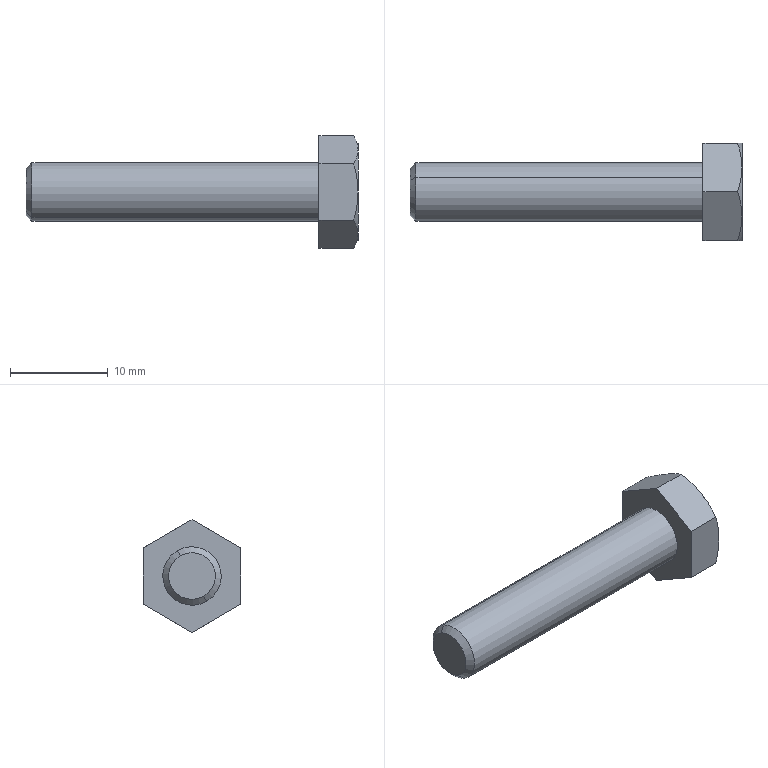Component | SolidWorks | Q1-A12-S21-Q1D.SLDASQ-1_Q1-RCB6-30-1 | 1 solid | 19 faces | box 34 x 10 x 11.55 mm | volume 1190 mm3 | plane 9 | cone 8 | cylinder 2 | commonest cylinder face diameters 6 x2
build123d program:
from build123d import *

# Parameters (mm, degrees)
SKETCH2_W          = 20
SKETCH2_H          = 20
CUT_EXTRUDE1_DEPTH = 4


with BuildPart() as part:
    # Sketch1 → Revolve1 (revolve)
    with BuildSketch(Plane.XY, mode=Mode.PRIVATE) as revolve1_sk:
        Polygon((-4, 0), (-4, 5), (-3.423, 6), (0, 6), (0, 3), (29.387, 3), (30, 2.386), (30, 0), align=None)
    revolve(revolve1_sk.sketch.rotate(Axis((30, 0, 0), (-1, 0, 0)), 270), axis=Axis((30, 0, 0), (-1, 0, 0)))

    # Sketch2 → Cut-Extrude1 (cut)
    with BuildSketch(Plane(origin=(-4, 0, 0), x_dir=(0, 0, -1), z_dir=(1, 0, 0))):
        Rectangle(SKETCH2_W, SKETCH2_H)
        Polygon((-5, -2.887), (0, -5.774), (5, -2.887), (5, 2.887), (0, 5.774), (-5, 2.887), align=None, mode=Mode.SUBTRACT)
    extrude(amount=CUT_EXTRUDE1_DEPTH, mode=Mode.SUBTRACT)


solid = part.part

# Placed as in the assembly
solid = solid.moved(Location((1985.5, 0, 156.25), (-90, 0, 180)))
STEP:
#1=COLOUR_RGB('',0.7922,0.8196,0.9333);
#2=FILL_AREA_STYLE_COLOUR('',#1);
#3=FILL_AREA_STYLE('',(#2));
#4=SURFACE_STYLE_FILL_AREA(#3);
#5=SURFACE_SIDE_STYLE('',(#4));
#6=SURFACE_STYLE_USAGE(.BOTH.,#5);
#7=PRESENTATION_STYLE_ASSIGNMENT((#6));
#8=CARTESIAN_POINT('',(76.988,-0.04698,6.07));
#9=VERTEX_POINT('',#8);
#10=CARTESIAN_POINT('',(76.988,0.04698,6.233));
#11=VERTEX_POINT('',#10);
#12=CARTESIAN_POINT('',(76.988,0.,6.152));
#13=DIRECTION('',(1.,-0.,-0.));
#14=DIRECTION('',(0.,-0.5,-0.866));
#15=AXIS2_PLACEMENT_3D('',#12,#13,#14);
#16=CIRCLE('',#15,0.09396);
#17=EDGE_CURVE('',#9,#11,#16,.T.);
#18=ORIENTED_EDGE('',*,*,#17,.T.);
#19=CARTESIAN_POINT('',(77.012,0.05906,6.254));
#20=VERTEX_POINT('',#19);
#21=CARTESIAN_POINT('',(76.988,0.04698,6.233));
#22=DIRECTION('',(0.7071,0.3536,0.6124));
#23=VECTOR('',#22,39.37);
#24=LINE('',#21,#23);
#25=EDGE_CURVE('',#11,#20,#24,.T.);
#26=ORIENTED_EDGE('',*,*,#25,.T.);
#27=CARTESIAN_POINT('',(77.012,-0.05906,6.049));
#28=VERTEX_POINT('',#27);
#29=CARTESIAN_POINT('',(77.012,0.,6.152));
#30=DIRECTION('',(1.,-0.,-0.));
#31=DIRECTION('',(0.,-0.5,-0.866));
#32=AXIS2_PLACEMENT_3D('',#29,#30,#31);
#33=CIRCLE('',#32,0.1181);
#34=EDGE_CURVE('',#28,#20,#33,.T.);
#35=ORIENTED_EDGE('',*,*,#34,.F.);
#36=CARTESIAN_POINT('',(76.988,-0.04698,6.07));
#37=DIRECTION('',(0.7071,-0.3536,-0.6124));
#38=VECTOR('',#37,39.37);
#39=LINE('',#36,#38);
#40=EDGE_CURVE('',#9,#28,#39,.T.);
#41=ORIENTED_EDGE('',*,*,#40,.F.);
#42=EDGE_LOOP('',(#18,#26,#35,#41));
#43=FACE_OUTER_BOUND('',#42,.T.);
#44=CARTESIAN_POINT('',(76.988,0.,6.152));
#45=DIRECTION('',(1.,-0.,-0.));
#46=DIRECTION('',(0.,-0.5,-0.866));
#47=AXIS2_PLACEMENT_3D('',#44,#45,#46);
#48=CONICAL_SURFACE('',#47,0.09396,0.7854);
#49=ADVANCED_FACE('',(#43),#48,.T.);
#50=ORIENTED_EDGE('',*,*,#34,.T.);
#51=CARTESIAN_POINT('',(78.169,0.05906,6.254));
#52=VERTEX_POINT('',#51);
#53=CARTESIAN_POINT('',(76.988,0.05906,6.254));
#54=DIRECTION('',(1.,-0.,-0.));
#55=VECTOR('',#54,39.37);
#56=LINE('',#53,#55);
#57=EDGE_CURVE('',#20,#52,#56,.T.);
#58=ORIENTED_EDGE('',*,*,#57,.T.);
#59=CARTESIAN_POINT('',(78.169,-0.05906,6.049));
#60=VERTEX_POINT('',#59);
#61=CARTESIAN_POINT('',(78.169,0.,6.152));
#62=DIRECTION('',(1.,-0.,-0.));
#63=DIRECTION('',(0.,-0.5,-0.866));
#64=AXIS2_PLACEMENT_3D('',#61,#62,#63);
#65=CIRCLE('',#64,0.1181);
#66=EDGE_CURVE('',#60,#52,#65,.T.);
#67=ORIENTED_EDGE('',*,*,#66,.F.);
#68=CARTESIAN_POINT('',(76.988,-0.05906,6.049));
#69=DIRECTION('',(1.,-0.,-0.));
#70=VECTOR('',#69,39.37);
#71=LINE('',#68,#70);
#72=EDGE_CURVE('',#28,#60,#71,.T.);
#73=ORIENTED_EDGE('',*,*,#72,.F.);
#74=EDGE_LOOP('',(#50,#58,#67,#73));
#75=FACE_OUTER_BOUND('',#74,.T.);
#76=CARTESIAN_POINT('',(76.988,0.,6.152));
#77=DIRECTION('',(1.,-0.,-0.));
#78=DIRECTION('',(0.,-0.5,-0.866));
#79=AXIS2_PLACEMENT_3D('',#76,#77,#78);
#80=CYLINDRICAL_SURFACE('',#79,0.1181);
#81=ADVANCED_FACE('',(#75),#80,.T.);
#82=CARTESIAN_POINT('',(78.169,0.1969,6.038));
#83=VERTEX_POINT('',#82);
#84=CARTESIAN_POINT('',(78.169,0.,5.924));
#85=VERTEX_POINT('',#84);
#86=CARTESIAN_POINT('',(78.169,0.1969,6.038));
#87=DIRECTION('',(-0.,-0.866,-0.5));
#88=VECTOR('',#87,39.37);
#89=LINE('',#86,#88);
#90=EDGE_CURVE('',#83,#85,#89,.T.);
#91=ORIENTED_EDGE('',*,*,#90,.T.);
#92=CARTESIAN_POINT('',(78.169,-0.1969,6.038));
#93=VERTEX_POINT('',#92);
#94=CARTESIAN_POINT('',(78.169,0.,5.924));
#95=DIRECTION('',(-0.,-0.866,0.5));
#96=VECTOR('',#95,39.37);
#97=LINE('',#94,#96);
#98=EDGE_CURVE('',#85,#93,#97,.T.);
#99=ORIENTED_EDGE('',*,*,#98,.T.);
#100=CARTESIAN_POINT('',(78.169,-0.1969,6.265));
#101=VERTEX_POINT('',#100);
#102=CARTESIAN_POINT('',(78.169,-0.1969,6.038));
#103=DIRECTION('',(-0.,-0.,1.));
#104=VECTOR('',#103,39.37);
#105=LINE('',#102,#104);
#106=EDGE_CURVE('',#93,#101,#105,.T.);
#107=ORIENTED_EDGE('',*,*,#106,.T.);
#108=CARTESIAN_POINT('',(78.169,0.,6.379));
#109=VERTEX_POINT('',#108);
#110=CARTESIAN_POINT('',(78.169,-0.1969,6.265));
#111=DIRECTION('',(0.,0.866,0.5));
#112=VECTOR('',#111,39.37);
#113=LINE('',#110,#112);
#114=EDGE_CURVE('',#101,#109,#113,.T.);
#115=ORIENTED_EDGE('',*,*,#114,.T.);
#116=CARTESIAN_POINT('',(78.169,0.1969,6.265));
#117=VERTEX_POINT('',#116);
#118=CARTESIAN_POINT('',(78.169,0.,6.379));
#119=DIRECTION('',(0.,0.866,-0.5));
#120=VECTOR('',#119,39.37);
#121=LINE('',#118,#120);
#122=EDGE_CURVE('',#109,#117,#121,.T.);
#123=ORIENTED_EDGE('',*,*,#122,.T.);
#124=CARTESIAN_POINT('',(78.169,0.1969,6.265));
#125=DIRECTION('',(0.,0.,-1.));
#126=VECTOR('',#125,39.37);
#127=LINE('',#124,#126);
#128=EDGE_CURVE('',#117,#83,#127,.T.);
#129=ORIENTED_EDGE('',*,*,#128,.T.);
#130=EDGE_LOOP('',(#91,#99,#107,#115,#123,#129));
#131=FACE_OUTER_BOUND('',#130,.T.);
#132=ORIENTED_EDGE('',*,*,#66,.T.);
#133=CARTESIAN_POINT('',(78.169,0.,6.152));
#134=DIRECTION('',(1.,-0.,-0.));
#135=DIRECTION('',(0.,-0.5,-0.866));
#136=AXIS2_PLACEMENT_3D('',#133,#134,#135);
#137=CIRCLE('',#136,0.1181);
#138=EDGE_CURVE('',#52,#60,#137,.T.);
#139=ORIENTED_EDGE('',*,*,#138,.T.);
#140=EDGE_LOOP('',(#132,#139));
#141=FACE_BOUND('',#140,.T.);
#142=CARTESIAN_POINT('',(78.169,0.2046,6.033));
#143=DIRECTION('',(1.,-0.,0.));
#144=DIRECTION('',(-0.,-0.5,-0.866));
#145=AXIS2_PLACEMENT_3D('',#142,#143,#144);
#146=PLANE('',#145);
#147=ADVANCED_FACE('',(#131,#141),#146,.F.);
#148=ORIENTED_EDGE('',*,*,#57,.F.);
#149=CARTESIAN_POINT('',(77.012,0.,6.152));
#150=DIRECTION('',(1.,-0.,-0.));
#151=DIRECTION('',(0.,-0.5,-0.866));
#152=AXIS2_PLACEMENT_3D('',#149,#150,#151);
#153=CIRCLE('',#152,0.1181);
#154=EDGE_CURVE('',#20,#28,#153,.T.);
#155=ORIENTED_EDGE('',*,*,#154,.T.);
#156=ORIENTED_EDGE('',*,*,#72,.T.);
#157=ORIENTED_EDGE('',*,*,#138,.F.);
#158=EDGE_LOOP('',(#148,#155,#156,#157));
#159=FACE_OUTER_BOUND('',#158,.T.);
#160=CARTESIAN_POINT('',(76.988,0.,6.152));
#161=DIRECTION('',(1.,-0.,-0.));
#162=DIRECTION('',(0.,-0.5,-0.866));
#163=AXIS2_PLACEMENT_3D('',#160,#161,#162);
#164=CYLINDRICAL_SURFACE('',#163,0.1181);
#165=ADVANCED_FACE('',(#159),#164,.T.);
#166=ORIENTED_EDGE('',*,*,#25,.F.);
#167=CARTESIAN_POINT('',(76.988,0.,6.152));
#168=DIRECTION('',(1.,-0.,-0.));
#169=DIRECTION('',(0.,-0.5,-0.866));
#170=AXIS2_PLACEMENT_3D('',#167,#168,#169);
#171=CIRCLE('',#170,0.09396);
#172=EDGE_CURVE('',#11,#9,#171,.T.);
#173=ORIENTED_EDGE('',*,*,#172,.T.);
#174=ORIENTED_EDGE('',*,*,#40,.T.);
#175=ORIENTED_EDGE('',*,*,#154,.F.);
#176=EDGE_LOOP('',(#166,#173,#174,#175));
#177=FACE_OUTER_BOUND('',#176,.T.);
#178=CARTESIAN_POINT('',(76.988,0.,6.152));
#179=DIRECTION('',(1.,-0.,-0.));
#180=DIRECTION('',(0.,-0.5,-0.866));
#181=AXIS2_PLACEMENT_3D('',#178,#179,#180);
#182=CONICAL_SURFACE('',#181,0.09396,0.7854);
#183=ADVANCED_FACE('',(#177),#182,.T.);
#184=ORIENTED_EDGE('',*,*,#17,.F.);
#185=ORIENTED_EDGE('',*,*,#172,.F.);
#186=EDGE_LOOP('',(#184,#185));
#187=FACE_OUTER_BOUND('',#186,.T.);
#188=CARTESIAN_POINT('',(76.988,0.08137,6.105));
#189=DIRECTION('',(1.,-0.,0.));
#190=DIRECTION('',(-0.,-0.5,-0.866));
#191=AXIS2_PLACEMENT_3D('',#188,#189,#190);
#192=PLANE('',#191);
#193=ADVANCED_FACE('',(#187),#192,.F.);
#194=CARTESIAN_POINT('',(78.309,-0.1969,6.038));
#195=VERTEX_POINT('',#194);
#196=CARTESIAN_POINT('',(78.169,-0.1969,6.038));
#197=DIRECTION('',(1.,-0.,-0.));
#198=VECTOR('',#197,39.37);
#199=LINE('',#196,#198);
#200=EDGE_CURVE('',#93,#195,#199,.T.);
#201=ORIENTED_EDGE('',*,*,#200,.F.);
#202=ORIENTED_EDGE('',*,*,#98,.F.);
#203=CARTESIAN_POINT('',(78.309,0.,5.924));
#204=VERTEX_POINT('',#203);
#205=CARTESIAN_POINT('',(78.169,0.,5.924));
#206=DIRECTION('',(1.,-0.,-0.));
#207=VECTOR('',#206,39.37);
#208=LINE('',#205,#207);
#209=EDGE_CURVE('',#85,#204,#208,.T.);
#210=ORIENTED_EDGE('',*,*,#209,.T.);
#211=CARTESIAN_POINT('',(78.327,-0.09843,5.981));
#212=VERTEX_POINT('',#211);
#213=CARTESIAN_POINT('',(78.327,-0.09843,5.981));
#214=CARTESIAN_POINT('',(78.327,-0.08178,5.971));
#215=CARTESIAN_POINT('',(78.325,-0.06491,5.962));
#216=CARTESIAN_POINT('',(78.319,-0.03204,5.943));
#217=CARTESIAN_POINT('',(78.314,-0.01592,5.933));
#218=CARTESIAN_POINT('',(78.309,0.,5.924));
#219=B_SPLINE_CURVE_WITH_KNOTS('',3,(#213,#214,#215,#216,#217,#218),.UNSPECIFIED.,.F.,.F.,(4,2,4),(0.008091,0.009552,0.01101),.UNSPECIFIED.);
#220=EDGE_CURVE('',#212,#204,#219,.T.);
#221=ORIENTED_EDGE('',*,*,#220,.F.);
#222=CARTESIAN_POINT('',(78.309,-0.1969,6.038));
#223=CARTESIAN_POINT('',(78.315,-0.1808,6.029));
#224=CARTESIAN_POINT('',(78.319,-0.1644,6.019));
#225=CARTESIAN_POINT('',(78.325,-0.1316,6.));
#226=CARTESIAN_POINT('',(78.327,-0.1151,5.991));
#227=CARTESIAN_POINT('',(78.327,-0.09843,5.981));
#228=B_SPLINE_CURVE_WITH_KNOTS('',3,(#222,#223,#224,#225,#226,#227),.UNSPECIFIED.,.F.,.F.,(4,2,4),(0.00517,0.006631,0.008091),.UNSPECIFIED.);
#229=EDGE_CURVE('',#195,#212,#228,.T.);
#230=ORIENTED_EDGE('',*,*,#229,.F.);
#231=EDGE_LOOP('',(#201,#202,#210,#221,#230));
#232=FACE_OUTER_BOUND('',#231,.T.);
#233=CARTESIAN_POINT('',(78.169,0.,5.924));
#234=DIRECTION('',(0.,0.5,0.866));
#235=DIRECTION('',(1.,-0.,-0.));
#236=AXIS2_PLACEMENT_3D('',#233,#234,#235);
#237=PLANE('',#236);
#238=ADVANCED_FACE('',(#232),#237,.F.);
#239=CARTESIAN_POINT('',(78.309,-0.1969,6.265));
#240=VERTEX_POINT('',#239);
#241=CARTESIAN_POINT('',(78.169,-0.1969,6.265));
#242=DIRECTION('',(1.,-0.,-0.));
#243=VECTOR('',#242,39.37);
#244=LINE('',#241,#243);
#245=EDGE_CURVE('',#101,#240,#244,.T.);
#246=ORIENTED_EDGE('',*,*,#245,.F.);
#247=ORIENTED_EDGE('',*,*,#106,.F.);
#248=ORIENTED_EDGE('',*,*,#200,.T.);
#249=CARTESIAN_POINT('',(78.327,-0.1969,6.152));
#250=VERTEX_POINT('',#249);
#251=CARTESIAN_POINT('',(78.327,-0.1969,6.152));
#252=CARTESIAN_POINT('',(78.327,-0.1969,6.142));
#253=CARTESIAN_POINT('',(78.326,-0.1969,6.132));
#254=CARTESIAN_POINT('',(78.325,-0.1969,6.113));
#255=CARTESIAN_POINT('',(78.324,-0.1969,6.104));
#256=CARTESIAN_POINT('',(78.319,-0.1969,6.075));
#257=CARTESIAN_POINT('',(78.315,-0.1969,6.056));
#258=CARTESIAN_POINT('',(78.309,-0.1969,6.038));
#259=B_SPLINE_CURVE_WITH_KNOTS('',3,(#251,#252,#253,#254,#255,#256,#257,#258),.UNSPECIFIED.,.F.,.F.,(4,2,2,4),(0.002921,0.003649,0.004376,0.005831),.UNSPECIFIED.);
#260=EDGE_CURVE('',#250,#195,#259,.T.);
#261=ORIENTED_EDGE('',*,*,#260,.F.);
#262=CARTESIAN_POINT('',(78.309,-0.1969,6.265));
#263=CARTESIAN_POINT('',(78.32,-0.1969,6.228));
#264=CARTESIAN_POINT('',(78.327,-0.1969,6.19));
#265=CARTESIAN_POINT('',(78.327,-0.1969,6.152));
#266=B_SPLINE_CURVE_WITH_KNOTS('',3,(#262,#263,#264,#265),.UNSPECIFIED.,.F.,.F.,(4,4),(0.00000024,0.002921),.UNSPECIFIED.);
#267=EDGE_CURVE('',#240,#250,#266,.T.);
#268=ORIENTED_EDGE('',*,*,#267,.F.);
#269=EDGE_LOOP('',(#246,#247,#248,#261,#268));
#270=FACE_OUTER_BOUND('',#269,.T.);
#271=CARTESIAN_POINT('',(78.169,-0.1969,6.038));
#272=DIRECTION('',(0.,1.,0.));
#273=DIRECTION('',(0.,0.,-1.));
#274=AXIS2_PLACEMENT_3D('',#271,#272,#273);
#275=PLANE('',#274);
#276=ADVANCED_FACE('',(#270),#275,.F.);
#277=CARTESIAN_POINT('',(78.309,0.,6.379));
#278=VERTEX_POINT('',#277);
#279=CARTESIAN_POINT('',(78.169,0.,6.379));
#280=DIRECTION('',(1.,-0.,-0.));
#281=VECTOR('',#280,39.37);
#282=LINE('',#279,#281);
#283=EDGE_CURVE('',#109,#278,#282,.T.);
#284=ORIENTED_EDGE('',*,*,#283,.F.);
#285=ORIENTED_EDGE('',*,*,#114,.F.);
#286=ORIENTED_EDGE('',*,*,#245,.T.);
#287=CARTESIAN_POINT('',(78.327,-0.09843,6.322));
#288=VERTEX_POINT('',#287);
#289=CARTESIAN_POINT('',(78.327,-0.09843,6.322));
#290=CARTESIAN_POINT('',(78.327,-0.1068,6.317));
#291=CARTESIAN_POINT('',(78.326,-0.1152,6.312));
#292=CARTESIAN_POINT('',(78.325,-0.1318,6.303));
#293=CARTESIAN_POINT('',(78.324,-0.14,6.298));
#294=CARTESIAN_POINT('',(78.319,-0.1646,6.284));
#295=CARTESIAN_POINT('',(78.315,-0.1808,6.274));
#296=CARTESIAN_POINT('',(78.309,-0.1969,6.265));
#297=B_SPLINE_CURVE_WITH_KNOTS('',3,(#289,#290,#291,#292,#293,#294,#295,#296),.UNSPECIFIED.,.F.,.F.,(4,2,2,4),(0.002921,0.003649,0.004376,0.005831),.UNSPECIFIED.);
#298=EDGE_CURVE('',#288,#240,#297,.T.);
#299=ORIENTED_EDGE('',*,*,#298,.F.);
#300=CARTESIAN_POINT('',(78.309,0.,6.379));
#301=CARTESIAN_POINT('',(78.32,-0.0322,6.36));
#302=CARTESIAN_POINT('',(78.327,-0.06489,6.341));
#303=CARTESIAN_POINT('',(78.327,-0.09843,6.322));
#304=B_SPLINE_CURVE_WITH_KNOTS('',3,(#300,#301,#302,#303),.UNSPECIFIED.,.F.,.F.,(4,4),(0.00000024,0.002921),.UNSPECIFIED.);
#305=EDGE_CURVE('',#278,#288,#304,.T.);
#306=ORIENTED_EDGE('',*,*,#305,.F.);
#307=EDGE_LOOP('',(#284,#285,#286,#299,#306));
#308=FACE_OUTER_BOUND('',#307,.T.);
#309=CARTESIAN_POINT('',(78.169,-0.1969,6.265));
#310=DIRECTION('',(0.,0.5,-0.866));
#311=DIRECTION('',(-0.,-0.866,-0.5));
#312=AXIS2_PLACEMENT_3D('',#309,#310,#311);
#313=PLANE('',#312);
#314=ADVANCED_FACE('',(#308),#313,.F.);
#315=CARTESIAN_POINT('',(78.309,0.1969,6.265));
#316=VERTEX_POINT('',#315);
#317=CARTESIAN_POINT('',(78.169,0.1969,6.265));
#318=DIRECTION('',(1.,-0.,-0.));
#319=VECTOR('',#318,39.37);
#320=LINE('',#317,#319);
#321=EDGE_CURVE('',#117,#316,#320,.T.);
#322=ORIENTED_EDGE('',*,*,#321,.F.);
#323=ORIENTED_EDGE('',*,*,#122,.F.);
#324=ORIENTED_EDGE('',*,*,#283,.T.);
#325=CARTESIAN_POINT('',(78.327,0.09843,6.322));
#326=VERTEX_POINT('',#325);
#327=CARTESIAN_POINT('',(78.327,0.09843,6.322));
#328=CARTESIAN_POINT('',(78.327,0.08179,6.332));
#329=CARTESIAN_POINT('',(78.325,0.06527,6.341));
#330=CARTESIAN_POINT('',(78.319,0.03241,6.36));
#331=CARTESIAN_POINT('',(78.315,0.01601,6.37));
#332=CARTESIAN_POINT('',(78.309,0.,6.379));
#333=B_SPLINE_CURVE_WITH_KNOTS('',3,(#327,#328,#329,#330,#331,#332),.UNSPECIFIED.,.F.,.F.,(4,2,4),(0.0156,0.01706,0.01852),.UNSPECIFIED.);
#334=EDGE_CURVE('',#326,#278,#333,.T.);
#335=ORIENTED_EDGE('',*,*,#334,.F.);
#336=CARTESIAN_POINT('',(78.309,0.1969,6.265));
#337=CARTESIAN_POINT('',(78.314,0.1809,6.274));
#338=CARTESIAN_POINT('',(78.319,0.1648,6.284));
#339=CARTESIAN_POINT('',(78.325,0.1319,6.303));
#340=CARTESIAN_POINT('',(78.327,0.1151,6.312));
#341=CARTESIAN_POINT('',(78.327,0.09843,6.322));
#342=B_SPLINE_CURVE_WITH_KNOTS('',3,(#336,#337,#338,#339,#340,#341),.UNSPECIFIED.,.F.,.F.,(4,2,4),(0.01267,0.01414,0.0156),.UNSPECIFIED.);
#343=EDGE_CURVE('',#316,#326,#342,.T.);
#344=ORIENTED_EDGE('',*,*,#343,.F.);
#345=EDGE_LOOP('',(#322,#323,#324,#335,#344));
#346=FACE_OUTER_BOUND('',#345,.T.);
#347=CARTESIAN_POINT('',(78.169,0.,6.379));
#348=DIRECTION('',(-0.,-0.5,-0.866));
#349=DIRECTION('',(-1.,0.,0.));
#350=AXIS2_PLACEMENT_3D('',#347,#348,#349);
#351=PLANE('',#350);
#352=ADVANCED_FACE('',(#346),#351,.F.);
#353=CARTESIAN_POINT('',(78.309,0.1969,6.038));
#354=VERTEX_POINT('',#353);
#355=CARTESIAN_POINT('',(78.169,0.1969,6.038));
#356=DIRECTION('',(1.,-0.,-0.));
#357=VECTOR('',#356,39.37);
#358=LINE('',#355,#357);
#359=EDGE_CURVE('',#83,#354,#358,.T.);
#360=ORIENTED_EDGE('',*,*,#359,.F.);
#361=ORIENTED_EDGE('',*,*,#128,.F.);
#362=ORIENTED_EDGE('',*,*,#321,.T.);
#363=CARTESIAN_POINT('',(78.327,0.1969,6.152));
#364=VERTEX_POINT('',#363);
#365=CARTESIAN_POINT('',(78.327,0.1969,6.152));
#366=CARTESIAN_POINT('',(78.327,0.1969,6.161));
#367=CARTESIAN_POINT('',(78.326,0.1969,6.171));
#368=CARTESIAN_POINT('',(78.325,0.1969,6.19));
#369=CARTESIAN_POINT('',(78.324,0.1969,6.2));
#370=CARTESIAN_POINT('',(78.319,0.1969,6.228));
#371=CARTESIAN_POINT('',(78.315,0.1969,6.247));
#372=CARTESIAN_POINT('',(78.309,0.1969,6.265));
#373=B_SPLINE_CURVE_WITH_KNOTS('',3,(#365,#366,#367,#368,#369,#370,#371,#372),.UNSPECIFIED.,.F.,.F.,(4,2,2,4),(0.002921,0.003649,0.004376,0.005831),.UNSPECIFIED.);
#374=EDGE_CURVE('',#364,#316,#373,.T.);
#375=ORIENTED_EDGE('',*,*,#374,.F.);
#376=CARTESIAN_POINT('',(78.309,0.1969,6.038));
#377=CARTESIAN_POINT('',(78.32,0.1969,6.075));
#378=CARTESIAN_POINT('',(78.327,0.1969,6.113));
#379=CARTESIAN_POINT('',(78.327,0.1969,6.152));
#380=B_SPLINE_CURVE_WITH_KNOTS('',3,(#376,#377,#378,#379),.UNSPECIFIED.,.F.,.F.,(4,4),(0.00000024,0.002921),.UNSPECIFIED.);
#381=EDGE_CURVE('',#354,#364,#380,.T.);
#382=ORIENTED_EDGE('',*,*,#381,.F.);
#383=EDGE_LOOP('',(#360,#361,#362,#375,#382));
#384=FACE_OUTER_BOUND('',#383,.T.);
#385=CARTESIAN_POINT('',(78.169,0.1969,6.265));
#386=DIRECTION('',(-0.,-1.,-0.));
#387=DIRECTION('',(-0.,-0.,1.));
#388=AXIS2_PLACEMENT_3D('',#385,#386,#387);
#389=PLANE('',#388);
#390=ADVANCED_FACE('',(#384),#389,.F.);
#391=ORIENTED_EDGE('',*,*,#209,.F.);
#392=ORIENTED_EDGE('',*,*,#90,.F.);
#393=ORIENTED_EDGE('',*,*,#359,.T.);
#394=CARTESIAN_POINT('',(78.327,0.09843,5.981));
#395=VERTEX_POINT('',#394);
#396=CARTESIAN_POINT('',(78.327,0.09843,5.981));
#397=CARTESIAN_POINT('',(78.327,0.1068,5.986));
#398=CARTESIAN_POINT('',(78.326,0.1152,5.991));
#399=CARTESIAN_POINT('',(78.325,0.1318,6.));
#400=CARTESIAN_POINT('',(78.324,0.14,6.005));
#401=CARTESIAN_POINT('',(78.319,0.1646,6.019));
#402=CARTESIAN_POINT('',(78.315,0.1808,6.029));
#403=CARTESIAN_POINT('',(78.309,0.1969,6.038));
#404=B_SPLINE_CURVE_WITH_KNOTS('',3,(#396,#397,#398,#399,#400,#401,#402,#403),.UNSPECIFIED.,.F.,.F.,(4,2,2,4),(0.002921,0.003649,0.004376,0.005831),.UNSPECIFIED.);
#405=EDGE_CURVE('',#395,#354,#404,.T.);
#406=ORIENTED_EDGE('',*,*,#405,.F.);
#407=CARTESIAN_POINT('',(78.309,0.,5.924));
#408=CARTESIAN_POINT('',(78.32,0.0322,5.943));
#409=CARTESIAN_POINT('',(78.327,0.06489,5.962));
#410=CARTESIAN_POINT('',(78.327,0.09843,5.981));
#411=B_SPLINE_CURVE_WITH_KNOTS('',3,(#407,#408,#409,#410),.UNSPECIFIED.,.F.,.F.,(4,4),(0.00000024,0.002921),.UNSPECIFIED.);
#412=EDGE_CURVE('',#204,#395,#411,.T.);
#413=ORIENTED_EDGE('',*,*,#412,.F.);
#414=EDGE_LOOP('',(#391,#392,#393,#406,#413));
#415=FACE_OUTER_BOUND('',#414,.T.);
#416=CARTESIAN_POINT('',(78.169,0.1969,6.038));
#417=DIRECTION('',(-0.,-0.5,0.866));
#418=DIRECTION('',(0.,0.866,0.5));
#419=AXIS2_PLACEMENT_3D('',#416,#417,#418);
#420=PLANE('',#419);
#421=ADVANCED_FACE('',(#415),#420,.F.);
#422=CARTESIAN_POINT('',(78.327,0.,6.152));
#423=DIRECTION('',(1.,-0.,-0.));
#424=DIRECTION('',(0.,-0.5,-0.866));
#425=AXIS2_PLACEMENT_3D('',#422,#423,#424);
#426=CIRCLE('',#425,0.1969);
#427=EDGE_CURVE('',#250,#212,#426,.T.);
#428=ORIENTED_EDGE('',*,*,#427,.F.);
#429=ORIENTED_EDGE('',*,*,#260,.T.);
#430=ORIENTED_EDGE('',*,*,#229,.T.);
#431=EDGE_LOOP('',(#428,#429,#430));
#432=FACE_OUTER_BOUND('',#431,.T.);
#433=CARTESIAN_POINT('',(78.304,0.,6.152));
#434=DIRECTION('',(-1.,0.,0.));
#435=DIRECTION('',(0.,0.5,0.866));
#436=AXIS2_PLACEMENT_3D('',#433,#434,#435);
#437=CONICAL_SURFACE('',#436,0.2362,1.047);
#438=ADVANCED_FACE('',(#432),#437,.T.);
#439=CARTESIAN_POINT('',(78.327,0.,6.152));
#440=DIRECTION('',(1.,-0.,-0.));
#441=DIRECTION('',(0.,-0.5,-0.866));
#442=AXIS2_PLACEMENT_3D('',#439,#440,#441);
#443=CIRCLE('',#442,0.1969);
#444=EDGE_CURVE('',#288,#250,#443,.T.);
#445=ORIENTED_EDGE('',*,*,#444,.F.);
#446=ORIENTED_EDGE('',*,*,#298,.T.);
#447=ORIENTED_EDGE('',*,*,#267,.T.);
#448=EDGE_LOOP('',(#445,#446,#447));
#449=FACE_OUTER_BOUND('',#448,.T.);
#450=CARTESIAN_POINT('',(78.304,0.,6.152));
#451=DIRECTION('',(-1.,0.,0.));
#452=DIRECTION('',(0.,0.5,0.866));
#453=AXIS2_PLACEMENT_3D('',#450,#451,#452);
#454=CONICAL_SURFACE('',#453,0.2362,1.047);
#455=ADVANCED_FACE('',(#449),#454,.T.);
#456=ORIENTED_EDGE('',*,*,#334,.T.);
#457=ORIENTED_EDGE('',*,*,#305,.T.);
#458=CARTESIAN_POINT('',(78.327,0.,6.152));
#459=DIRECTION('',(1.,-0.,-0.));
#460=DIRECTION('',(0.,-0.5,-0.866));
#461=AXIS2_PLACEMENT_3D('',#458,#459,#460);
#462=CIRCLE('',#461,0.1969);
#463=EDGE_CURVE('',#326,#288,#462,.T.);
#464=ORIENTED_EDGE('',*,*,#463,.F.);
#465=EDGE_LOOP('',(#456,#457,#464));
#466=FACE_OUTER_BOUND('',#465,.T.);
#467=CARTESIAN_POINT('',(78.304,0.,6.152));
#468=DIRECTION('',(-1.,0.,0.));
#469=DIRECTION('',(0.,0.5,0.866));
#470=AXIS2_PLACEMENT_3D('',#467,#468,#469);
#471=CONICAL_SURFACE('',#470,0.2362,1.047);
#472=ADVANCED_FACE('',(#466),#471,.T.);
#473=ORIENTED_EDGE('',*,*,#374,.T.);
#474=ORIENTED_EDGE('',*,*,#343,.T.);
#475=CARTESIAN_POINT('',(78.327,0.,6.152));
#476=DIRECTION('',(1.,-0.,-0.));
#477=DIRECTION('',(0.,-0.5,-0.866));
#478=AXIS2_PLACEMENT_3D('',#475,#476,#477);
#479=CIRCLE('',#478,0.1969);
#480=EDGE_CURVE('',#364,#326,#479,.T.);
#481=ORIENTED_EDGE('',*,*,#480,.F.);
#482=EDGE_LOOP('',(#473,#474,#481));
#483=FACE_OUTER_BOUND('',#482,.T.);
#484=CARTESIAN_POINT('',(78.304,0.,6.152));
#485=DIRECTION('',(-1.,0.,0.));
#486=DIRECTION('',(0.,0.5,0.866));
#487=AXIS2_PLACEMENT_3D('',#484,#485,#486);
#488=CONICAL_SURFACE('',#487,0.2362,1.047);
#489=ADVANCED_FACE('',(#483),#488,.T.);
#490=CARTESIAN_POINT('',(78.327,0.,6.152));
#491=DIRECTION('',(1.,-0.,-0.));
#492=DIRECTION('',(0.,-0.5,-0.866));
#493=AXIS2_PLACEMENT_3D('',#490,#491,#492);
#494=CIRCLE('',#493,0.1969);
#495=EDGE_CURVE('',#212,#395,#494,.T.);
#496=ORIENTED_EDGE('',*,*,#495,.F.);
#497=ORIENTED_EDGE('',*,*,#220,.T.);
#498=ORIENTED_EDGE('',*,*,#412,.T.);
#499=EDGE_LOOP('',(#496,#497,#498));
#500=FACE_OUTER_BOUND('',#499,.T.);
#501=CARTESIAN_POINT('',(78.304,0.,6.152));
#502=DIRECTION('',(-1.,0.,0.));
#503=DIRECTION('',(0.,0.5,0.866));
#504=AXIS2_PLACEMENT_3D('',#501,#502,#503);
#505=CONICAL_SURFACE('',#504,0.2362,1.047);
#506=ADVANCED_FACE('',(#500),#505,.T.);
#507=ORIENTED_EDGE('',*,*,#495,.T.);
#508=CARTESIAN_POINT('',(78.327,0.,6.152));
#509=DIRECTION('',(1.,-0.,-0.));
#510=DIRECTION('',(0.,-0.5,-0.866));
#511=AXIS2_PLACEMENT_3D('',#508,#509,#510);
#512=CIRCLE('',#511,0.1969);
#513=EDGE_CURVE('',#395,#364,#512,.T.);
#514=ORIENTED_EDGE('',*,*,#513,.T.);
#515=ORIENTED_EDGE('',*,*,#480,.T.);
#516=ORIENTED_EDGE('',*,*,#463,.T.);
#517=ORIENTED_EDGE('',*,*,#444,.T.);
#518=ORIENTED_EDGE('',*,*,#427,.T.);
#519=EDGE_LOOP('',(#507,#514,#515,#516,#517,#518));
#520=FACE_OUTER_BOUND('',#519,.T.);
#521=CARTESIAN_POINT('',(78.327,0.,6.152));
#522=DIRECTION('',(-1.,0.,0.));
#523=DIRECTION('',(0.,0.5,0.866));
#524=AXIS2_PLACEMENT_3D('',#521,#522,#523);
#525=PLANE('',#524);
#526=ADVANCED_FACE('',(#520),#525,.F.);
#527=ORIENTED_EDGE('',*,*,#405,.T.);
#528=ORIENTED_EDGE('',*,*,#381,.T.);
#529=ORIENTED_EDGE('',*,*,#513,.F.);
#530=EDGE_LOOP('',(#527,#528,#529));
#531=FACE_OUTER_BOUND('',#530,.T.);
#532=CARTESIAN_POINT('',(78.304,0.,6.152));
#533=DIRECTION('',(-1.,0.,0.));
#534=DIRECTION('',(0.,0.5,0.866));
#535=AXIS2_PLACEMENT_3D('',#532,#533,#534);
#536=CONICAL_SURFACE('',#535,0.2362,1.047);
#537=ADVANCED_FACE('',(#531),#536,.T.);
#538=CLOSED_SHELL('',(#49,#81,#147,#165,#183,#193,#238,#276,#314,#352,#390,#421,#438,#455,#472,#489,#506,#526,#537));
#539=MANIFOLD_SOLID_BREP('',#538);
#540=STYLED_ITEM('',(#7),#539);
#541=(LENGTH_UNIT()NAMED_UNIT(*)SI_UNIT($,.METRE.));
#542=LENGTH_MEASURE_WITH_UNIT(LENGTH_MEASURE(0.0254),#541);
#543=DIMENSIONAL_EXPONENTS(1.,0.,0.,0.,0.,0.,0.);
#544=(CONVERSION_BASED_UNIT('',#542)LENGTH_UNIT()NAMED_UNIT(#543));
#545=UNCERTAINTY_MEASURE_WITH_UNIT(LENGTH_MEASURE(0.00001),#544,'','');
#546=(NAMED_UNIT(*)PLANE_ANGLE_UNIT()SI_UNIT($,.RADIAN.));
#547=(NAMED_UNIT(*)SI_UNIT($,.STERADIAN.)SOLID_ANGLE_UNIT());
#548=(GEOMETRIC_REPRESENTATION_CONTEXT(3)GLOBAL_UNCERTAINTY_ASSIGNED_CONTEXT((#545))GLOBAL_UNIT_ASSIGNED_CONTEXT((#544,#546,#547))REPRESENTATION_CONTEXT('',''));
#549=MECHANICAL_DESIGN_GEOMETRIC_PRESENTATION_REPRESENTATION('',(#540),#548);
#550=CARTESIAN_POINT('',(0.,0.,0.));
#551=DIRECTION('',(0.,0.,1.));
#552=DIRECTION('',(1.,0.,0.));
#553=AXIS2_PLACEMENT_3D('',#550,#551,#552);
#554=(LENGTH_UNIT()NAMED_UNIT(*)SI_UNIT($,.METRE.));
#555=LENGTH_MEASURE_WITH_UNIT(LENGTH_MEASURE(0.0254),#554);
#556=DIMENSIONAL_EXPONENTS(1.,0.,0.,0.,0.,0.,0.);
#557=(CONVERSION_BASED_UNIT('',#555)LENGTH_UNIT()NAMED_UNIT(#556));
#558=UNCERTAINTY_MEASURE_WITH_UNIT(LENGTH_MEASURE(0.00001),#557,'','');
#559=(NAMED_UNIT(*)PLANE_ANGLE_UNIT()SI_UNIT($,.RADIAN.));
#560=(NAMED_UNIT(*)SI_UNIT($,.STERADIAN.)SOLID_ANGLE_UNIT());
#561=(GEOMETRIC_REPRESENTATION_CONTEXT(3)GLOBAL_UNCERTAINTY_ASSIGNED_CONTEXT((#558))GLOBAL_UNIT_ASSIGNED_CONTEXT((#557,#559,#560))REPRESENTATION_CONTEXT('',''));
#562=ADVANCED_BREP_SHAPE_REPRESENTATION('',(#539,#553),#561);
#563=PRESENTATION_LAYER_ASSIGNMENT('','',(#540));